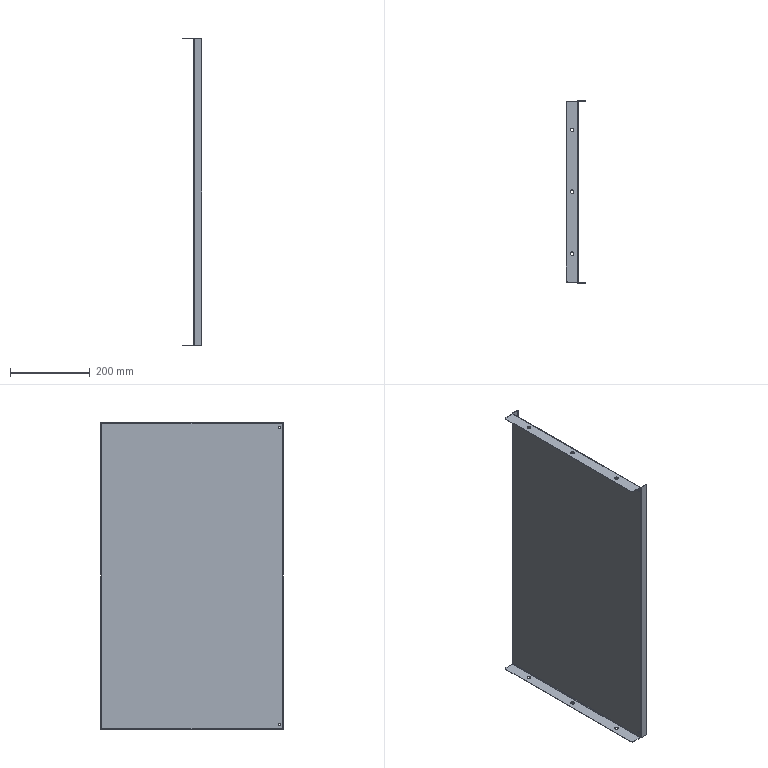Component | SolidWorks | MiddleConnectingPlate-1_MiddleUpperConnectingPlate-1 | 1 solid | 62 faces | volume 324805 mm3 | plane 34 | cylinder 28 | commonest cylinder face diameters 9 x12 6 x4 3.6 x4 2 x4 10 x4 | material 304